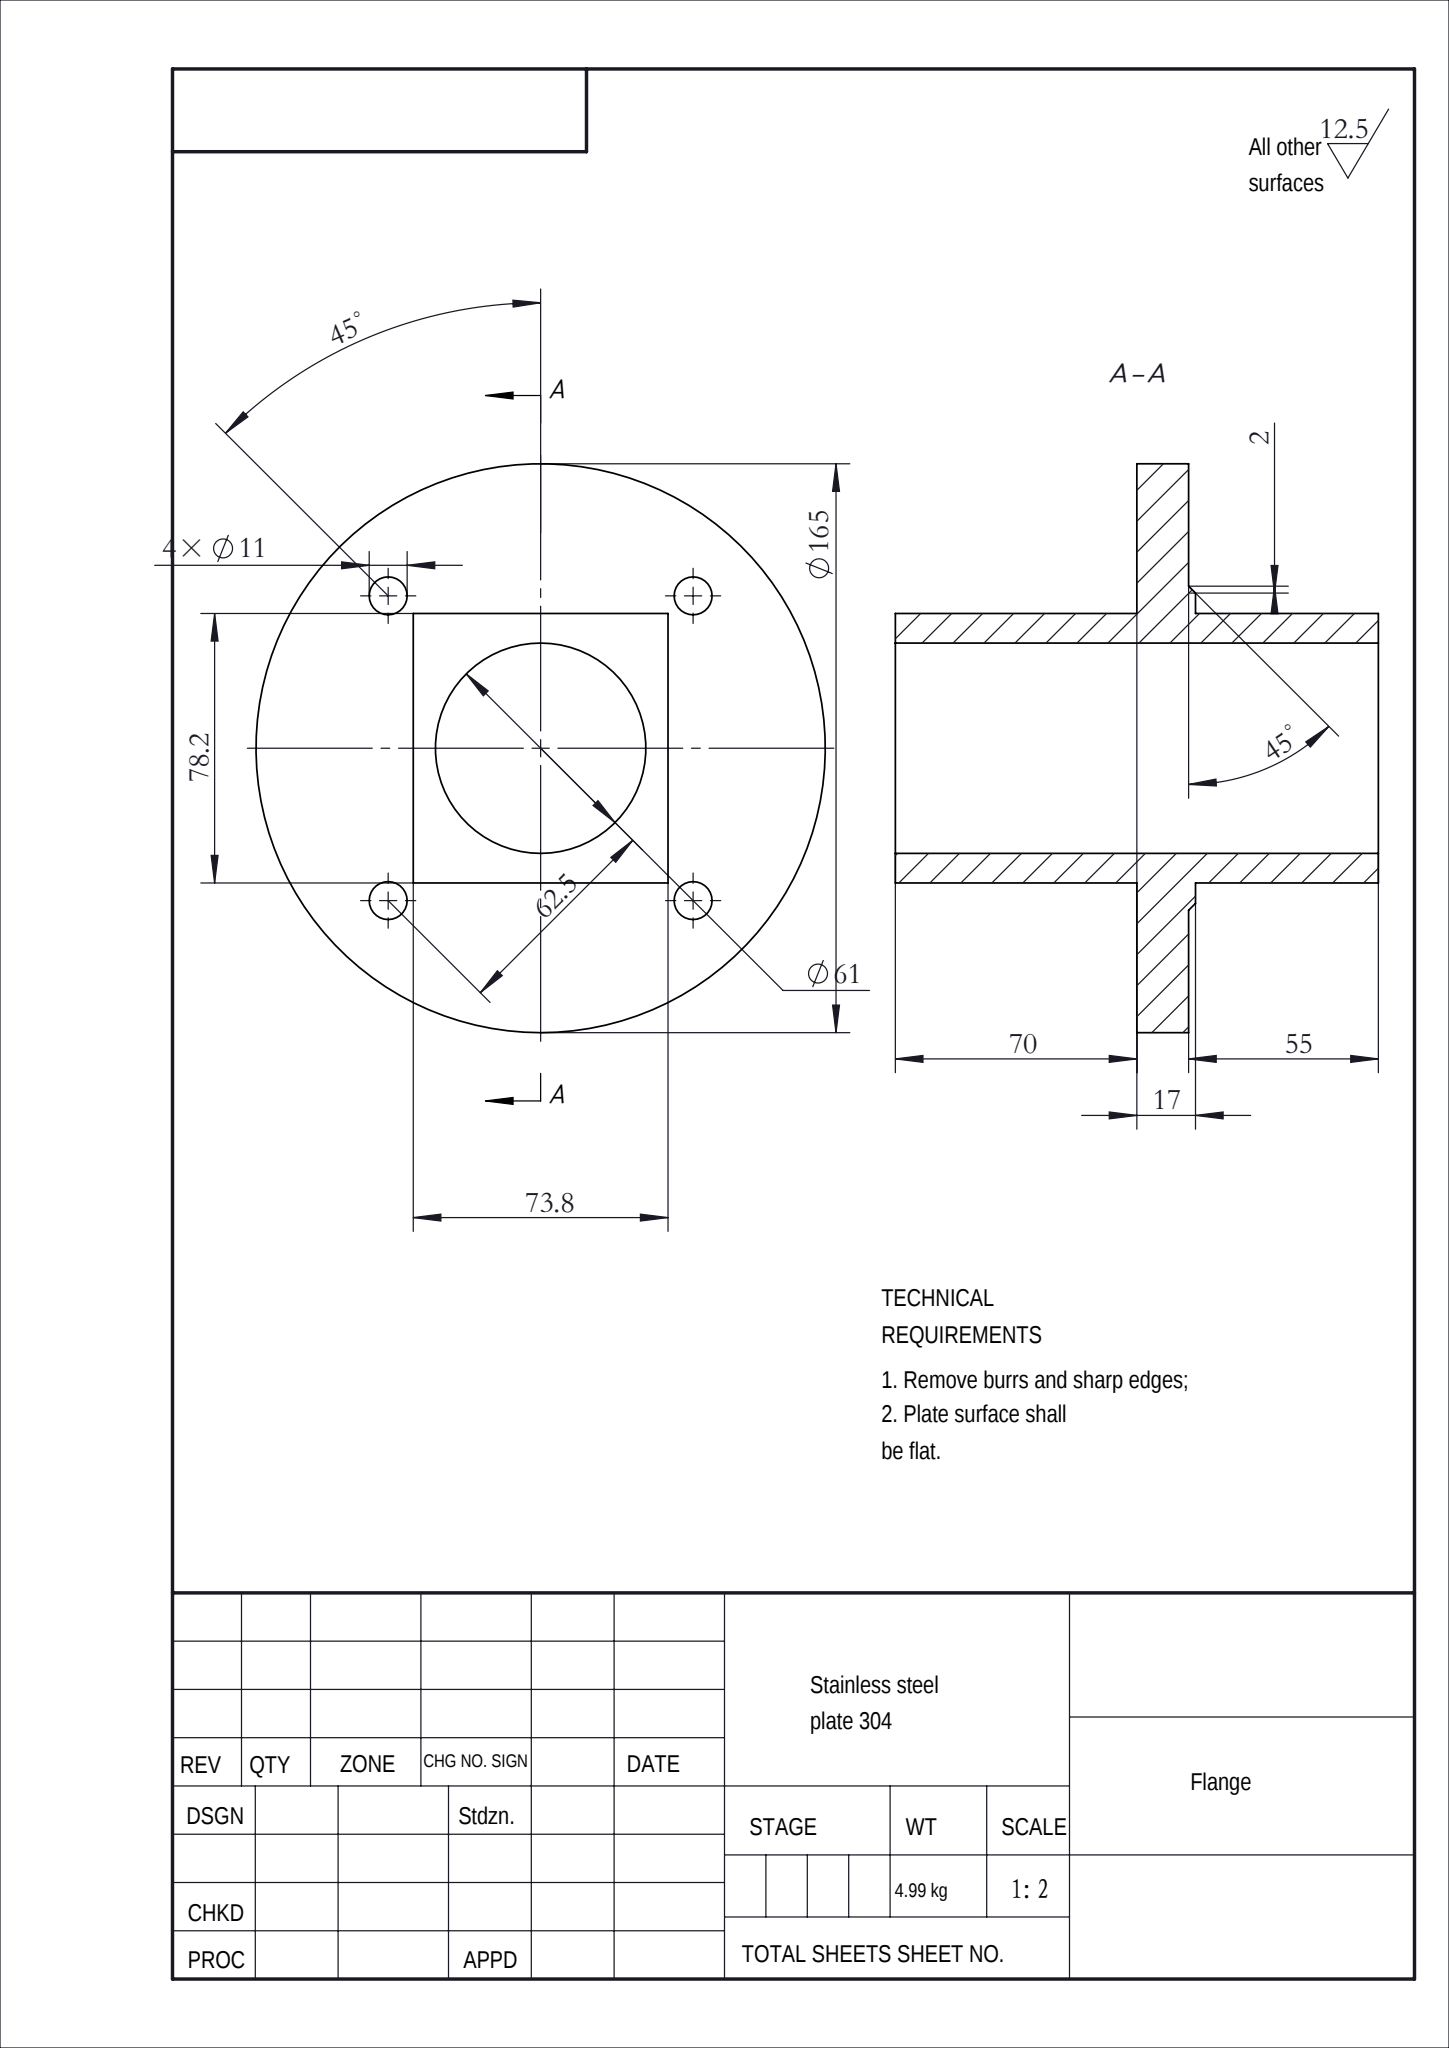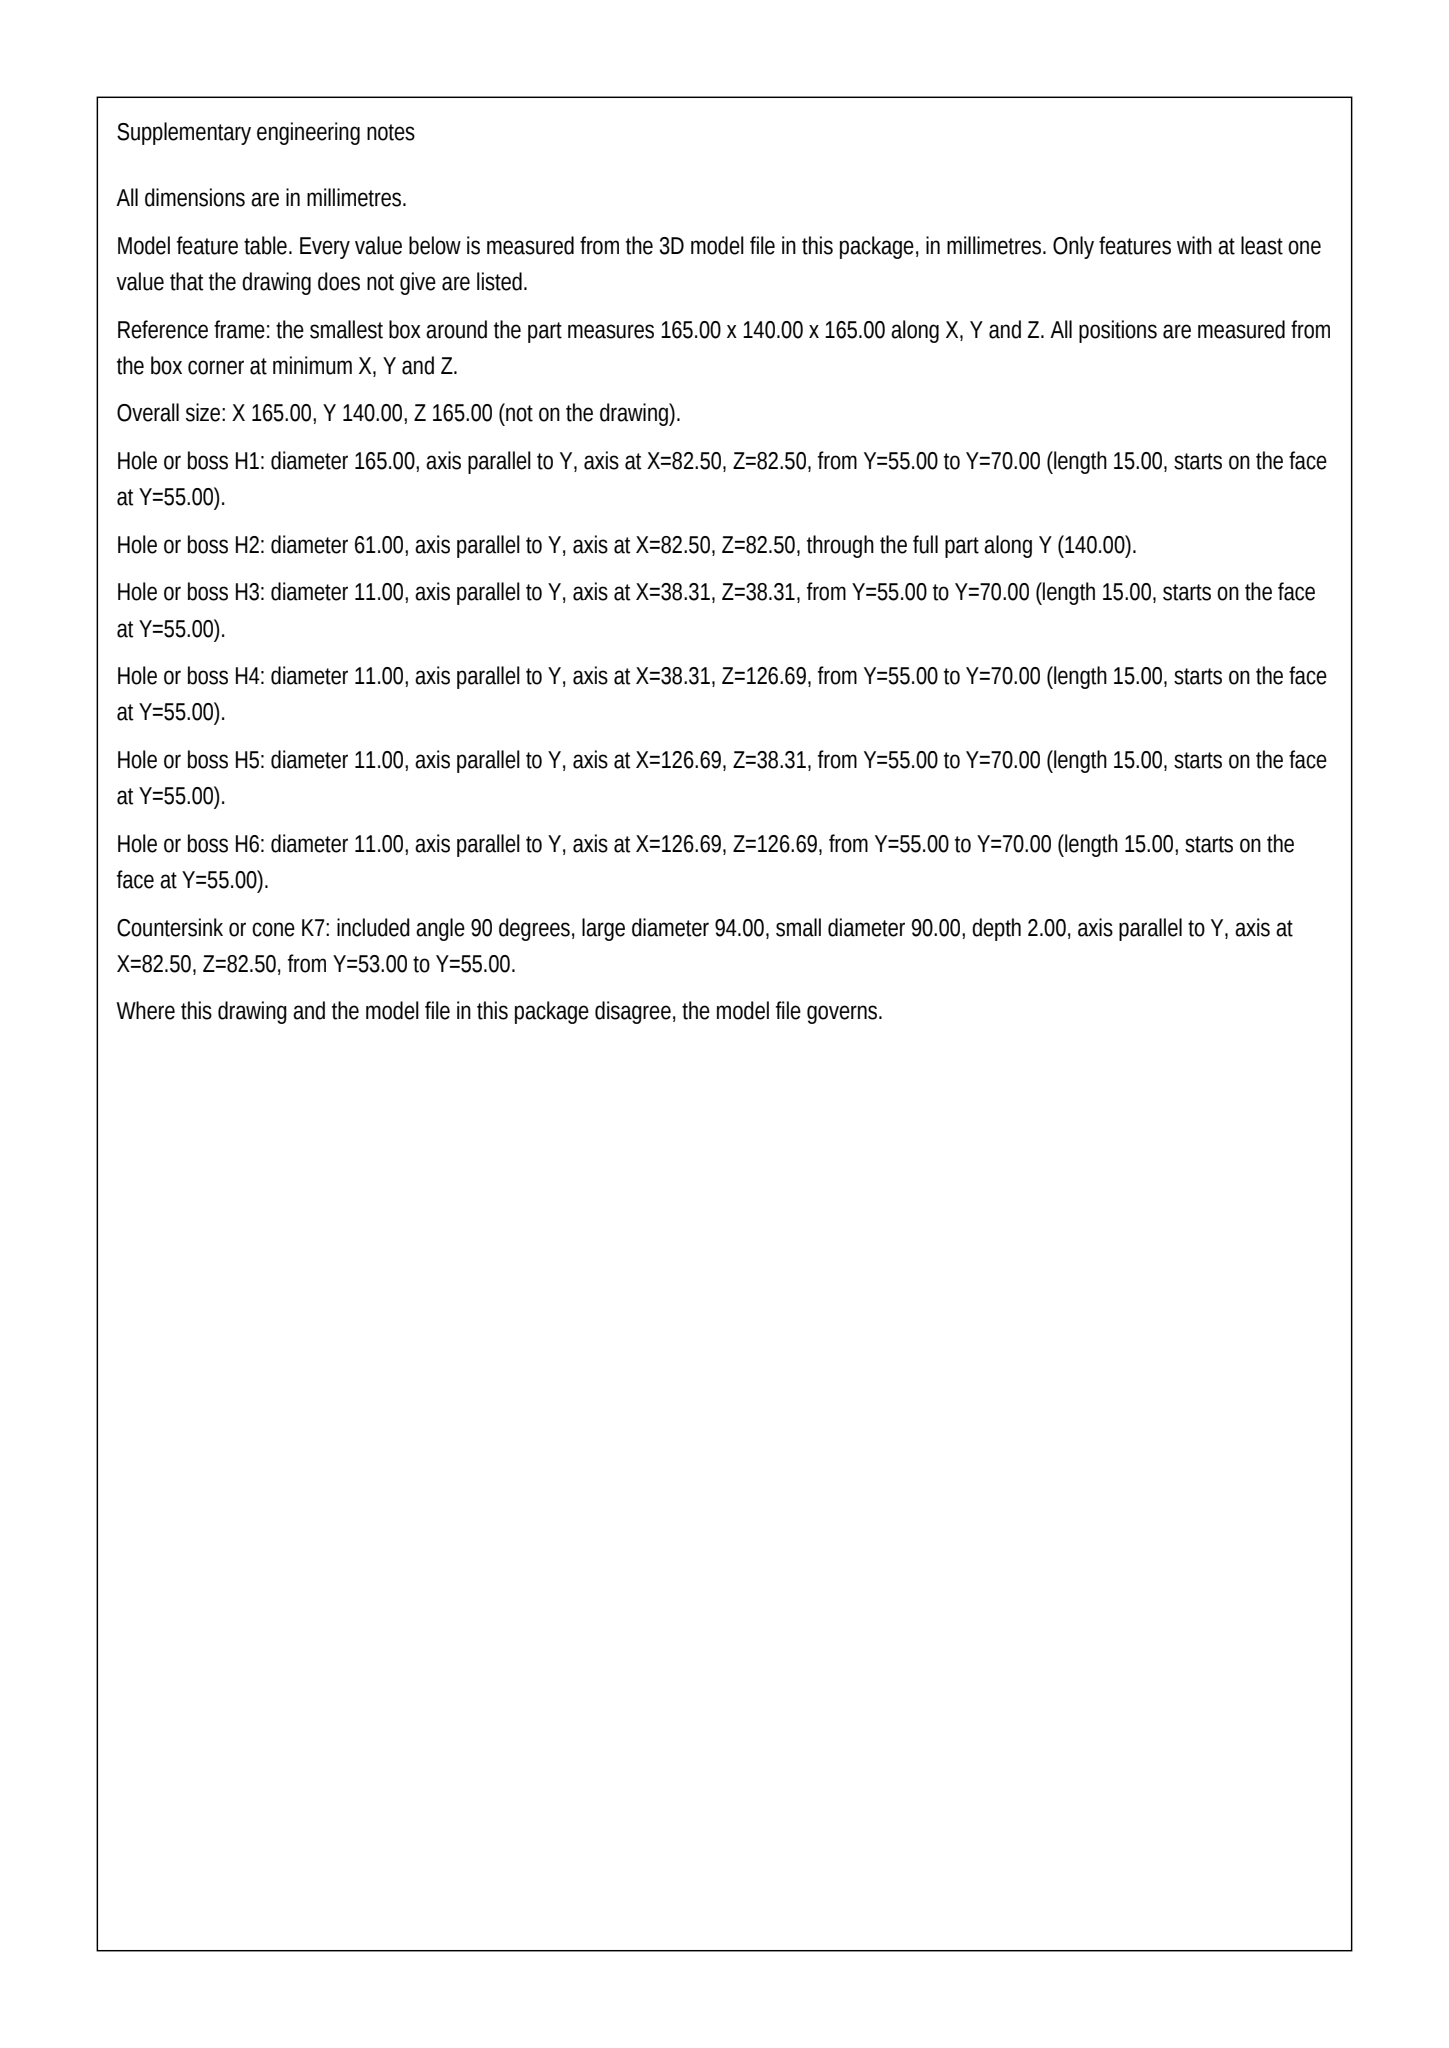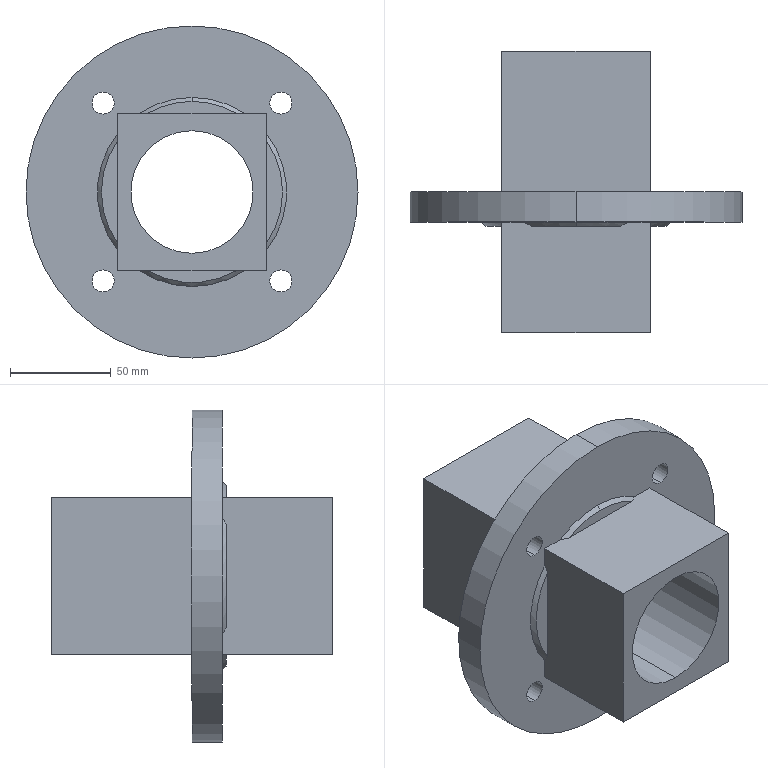Part | SolidWorks | material Stainless steel plate 304 | 1 solid | 33 faces | box 165 x 140 x 165 mm | volume 629628 mm3 | plane 16 | cylinder 12 | cone 5 | commonest cylinder face diameters 11 x8 61 x2 165 x2